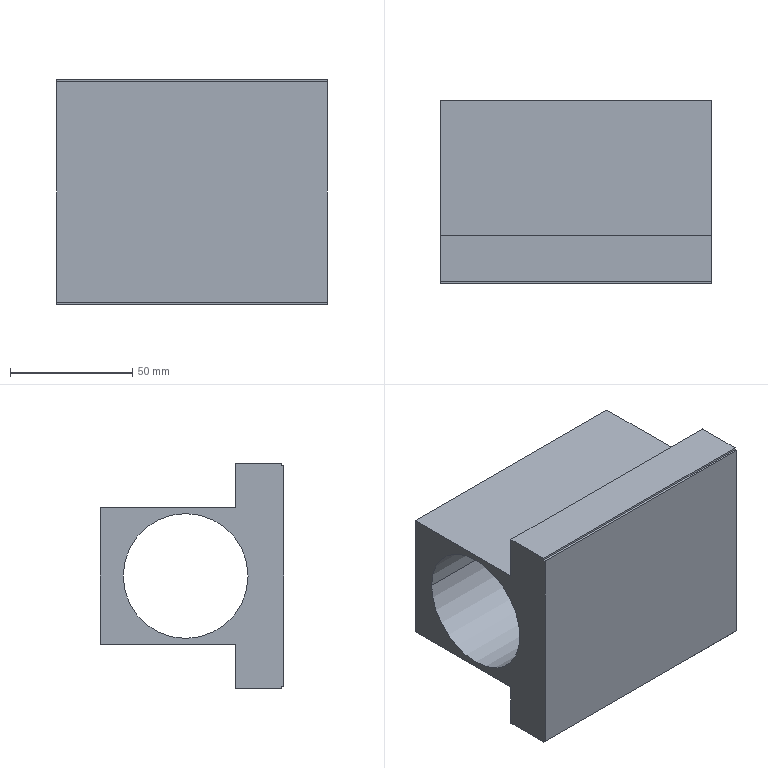Component | SolidWorks | ConnectingSeat-1 | 1 solid | 34 faces | box 111 x 75.24 x 92.14 mm | volume 314296 mm3 | plane 20 | cylinder 14 | commonest cylinder face diameters 8 x8 5.551 x4 51.14 x2
build123d program:
from build123d import *

# Parameters (mm, degrees)
BOSS_EXTRUDE1_DEPTH  = 111
SKETCH4_R            = 18.564
CUT_EXTRUDE1_2_DEPTH = 111
SKETCH5_W            = 55.24
SKETCH5_H            = 35.775
CUT_EXTRUDE2_DEPTH   = 171
SKETCH6_R            = 25.57
CUT_EXTRUDE3_DEPTH   = 115
SKETCH7_R            = 25.57
BOSS_EXTRUDE2_DEPTH  = 111
SKETCH9_R            = 4
CUT_EXTRUDE4_DEPTH   = 13.5
SKETCH10_R           = 2.776
CUT_EXTRUDE5_DEPTH   = 13.5
SKETCH1_W            = 1
SKETCH1_H            = 1.15
CUT_EXTRUDE1_DEPTH   = 133.269


with BuildPart() as part:
    # Sketch3 → Boss-Extrude1 (new body)
    with BuildSketch(Plane.ZY.offset(277)):
        Polygon((-20, -46.072), (-20, 46.072), (-0.1784, 46.072), (-0.1784, 27.887), (55.24, 27.887), (55.24, -27.887), (-0.1784, -27.887), (-0.1784, -46.072), align=None)
    extrude(amount=-BOSS_EXTRUDE1_DEPTH)

    # Sketch4 → Cut-Extrude1_2 (cut)
    with BuildSketch(Plane.ZY.offset(277)):
        with Locations((20.219, 0)):
            Circle(SKETCH4_R)
    extrude(amount=-CUT_EXTRUDE1_2_DEPTH, mode=Mode.SUBTRACT)

    # Sketch5 → Cut-Extrude2 (cut)
    with BuildSketch(Plane(origin=(-166, 0, 0), x_dir=(0, 0, -1), z_dir=(1, 0, 0))):
        with Locations((-17.62, 0)):
            Rectangle(SKETCH5_W, SKETCH5_H)
    extrude(amount=-CUT_EXTRUDE2_DEPTH, mode=Mode.SUBTRACT)

    # Sketch6 → Cut-Extrude3 (cut)
    with BuildSketch(Plane(origin=(-166, 0, 0), x_dir=(0, 0, -1), z_dir=(1, 0, 0))):
        with Locations((-20.219, 0)):
            Circle(SKETCH6_R)
    extrude(amount=-CUT_EXTRUDE3_DEPTH, mode=Mode.SUBTRACT)

    # Sketch7 → Boss-Extrude2 (add)
    with BuildSketch(Plane(origin=(-166, 0, 0), x_dir=(0, 0, -1), z_dir=(1, 0, 0))):
        Polygon((-55.24, 27.887), (-55.24, -27.887), (0.1784, -27.887), (0.1784, -46.072), (20, -46.072), (20, 46.072), (0.1784, 46.072), (0.1784, 27.887), align=None)
        with Locations((-20.219, 0)):
            Circle(SKETCH7_R, mode=Mode.SUBTRACT)
    extrude(amount=-BOSS_EXTRUDE2_DEPTH)

    # Sketch9 → Cut-Extrude4 (cut)
    with BuildSketch(Plane.XY.offset(-0.1784)):
        with Locations((-256.037, 36.566)):
            Circle(SKETCH9_R)
        with Locations((-186.382, 36.566)):
            Circle(SKETCH9_R)
        with Locations(Location((-186.382, -36.566, 0), (0, 0, 180))):
            Circle(SKETCH9_R)
        with Locations(Location((-256.037, -36.566, 0), (0, 0, 180))):
            Circle(SKETCH9_R)
    extrude(amount=-CUT_EXTRUDE4_DEPTH, mode=Mode.SUBTRACT)

    # Sketch10 → Cut-Extrude5 (cut)
    with BuildSketch(Plane.XY.offset(-0.1784)):
        with Locations((-221.326, 36.732)):
            Circle(SKETCH10_R)
        with Locations(Location((-221.326, -36.732, 0), (0, 0, 180))):
            Circle(SKETCH10_R)
    extrude(amount=-CUT_EXTRUDE5_DEPTH, mode=Mode.SUBTRACT)

    # Sketch1 → Cut-Extrude1 (cut, through all)
    with BuildSketch(Plane(origin=(-166, 0, 0), x_dir=(0, 0, -1), z_dir=(1, 0, 0))):
        with Locations((19.6, -45.825)):
            Rectangle(SKETCH1_W, SKETCH1_H)
        with Locations((19.6, 45.825)):
            Rectangle(SKETCH1_W, SKETCH1_H)
    extrude(amount=-CUT_EXTRUDE1_DEPTH, mode=Mode.SUBTRACT)


solid = part.part

# Placed as in the assembly
solid = solid.moved(Location((0, 40, 0), (-90, 0, 0)))
STEP:
#1=CARTESIAN_POINT('',(-8.823,1.036,1.446));
#2=VERTEX_POINT('',#1);
#3=CARTESIAN_POINT('',(-8.604,1.036,1.446));
#4=VERTEX_POINT('',#3);
#5=CARTESIAN_POINT('',(-8.714,1.036,1.446));
#6=DIRECTION('',(0.,1.,0.));
#7=DIRECTION('',(-1.,0.,0.));
#8=AXIS2_PLACEMENT_3D('',#5,#6,#7);
#9=CIRCLE('',#8,0.1093);
#10=EDGE_CURVE('',#2,#4,#9,.T.);
#11=ORIENTED_EDGE('',*,*,#10,.F.);
#12=CARTESIAN_POINT('',(-8.823,1.568,1.446));
#13=VERTEX_POINT('',#12);
#14=CARTESIAN_POINT('',(-8.823,1.036,1.446));
#15=DIRECTION('',(0.,1.,0.));
#16=VECTOR('',#15,39.37);
#17=LINE('',#14,#16);
#18=EDGE_CURVE('',#2,#13,#17,.T.);
#19=ORIENTED_EDGE('',*,*,#18,.T.);
#20=CARTESIAN_POINT('',(-8.604,1.568,1.446));
#21=VERTEX_POINT('',#20);
#22=CARTESIAN_POINT('',(-8.714,1.568,1.446));
#23=DIRECTION('',(0.,1.,0.));
#24=DIRECTION('',(-1.,0.,0.));
#25=AXIS2_PLACEMENT_3D('',#22,#23,#24);
#26=CIRCLE('',#25,0.1093);
#27=EDGE_CURVE('',#13,#21,#26,.T.);
#28=ORIENTED_EDGE('',*,*,#27,.T.);
#29=CARTESIAN_POINT('',(-8.604,1.036,1.446));
#30=DIRECTION('',(0.,1.,0.));
#31=VECTOR('',#30,39.37);
#32=LINE('',#29,#31);
#33=EDGE_CURVE('',#4,#21,#32,.T.);
#34=ORIENTED_EDGE('',*,*,#33,.F.);
#35=EDGE_LOOP('',(#11,#19,#28,#34));
#36=FACE_OUTER_BOUND('',#35,.T.);
#37=CARTESIAN_POINT('',(-8.714,1.036,1.446));
#38=DIRECTION('',(0.,1.,0.));
#39=DIRECTION('',(1.,0.,0.));
#40=AXIS2_PLACEMENT_3D('',#37,#38,#39);
#41=CYLINDRICAL_SURFACE('',#40,0.1093);
#42=ADVANCED_FACE('',(#36),#41,.F.);
#43=CARTESIAN_POINT('',(-8.823,1.036,-1.446));
#44=VERTEX_POINT('',#43);
#45=CARTESIAN_POINT('',(-8.604,1.036,-1.446));
#46=VERTEX_POINT('',#45);
#47=CARTESIAN_POINT('',(-8.714,1.036,-1.446));
#48=DIRECTION('',(0.,1.,0.));
#49=DIRECTION('',(1.,0.,0.));
#50=AXIS2_PLACEMENT_3D('',#47,#48,#49);
#51=CIRCLE('',#50,0.1093);
#52=EDGE_CURVE('',#44,#46,#51,.T.);
#53=ORIENTED_EDGE('',*,*,#52,.F.);
#54=CARTESIAN_POINT('',(-8.823,1.568,-1.446));
#55=VERTEX_POINT('',#54);
#56=CARTESIAN_POINT('',(-8.823,1.036,-1.446));
#57=DIRECTION('',(0.,1.,0.));
#58=VECTOR('',#57,39.37);
#59=LINE('',#56,#58);
#60=EDGE_CURVE('',#44,#55,#59,.T.);
#61=ORIENTED_EDGE('',*,*,#60,.T.);
#62=CARTESIAN_POINT('',(-8.604,1.568,-1.446));
#63=VERTEX_POINT('',#62);
#64=CARTESIAN_POINT('',(-8.714,1.568,-1.446));
#65=DIRECTION('',(0.,1.,0.));
#66=DIRECTION('',(1.,0.,0.));
#67=AXIS2_PLACEMENT_3D('',#64,#65,#66);
#68=CIRCLE('',#67,0.1093);
#69=EDGE_CURVE('',#55,#63,#68,.T.);
#70=ORIENTED_EDGE('',*,*,#69,.T.);
#71=CARTESIAN_POINT('',(-8.604,1.036,-1.446));
#72=DIRECTION('',(0.,1.,0.));
#73=VECTOR('',#72,39.37);
#74=LINE('',#71,#73);
#75=EDGE_CURVE('',#46,#63,#74,.T.);
#76=ORIENTED_EDGE('',*,*,#75,.F.);
#77=EDGE_LOOP('',(#53,#61,#70,#76));
#78=FACE_OUTER_BOUND('',#77,.T.);
#79=CARTESIAN_POINT('',(-8.714,1.036,-1.446));
#80=DIRECTION('',(0.,1.,0.));
#81=DIRECTION('',(1.,0.,0.));
#82=AXIS2_PLACEMENT_3D('',#79,#80,#81);
#83=CYLINDRICAL_SURFACE('',#82,0.1093);
#84=ADVANCED_FACE('',(#78),#83,.F.);
#85=CARTESIAN_POINT('',(-10.238,1.036,1.44));
#86=VERTEX_POINT('',#85);
#87=CARTESIAN_POINT('',(-9.923,1.036,1.44));
#88=VERTEX_POINT('',#87);
#89=CARTESIAN_POINT('',(-10.08,1.036,1.44));
#90=DIRECTION('',(0.,1.,0.));
#91=DIRECTION('',(-1.,0.,0.));
#92=AXIS2_PLACEMENT_3D('',#89,#90,#91);
#93=CIRCLE('',#92,0.1575);
#94=EDGE_CURVE('',#86,#88,#93,.T.);
#95=ORIENTED_EDGE('',*,*,#94,.F.);
#96=CARTESIAN_POINT('',(-10.238,1.568,1.44));
#97=VERTEX_POINT('',#96);
#98=CARTESIAN_POINT('',(-10.238,1.036,1.44));
#99=DIRECTION('',(0.,1.,0.));
#100=VECTOR('',#99,39.37);
#101=LINE('',#98,#100);
#102=EDGE_CURVE('',#86,#97,#101,.T.);
#103=ORIENTED_EDGE('',*,*,#102,.T.);
#104=CARTESIAN_POINT('',(-9.923,1.568,1.44));
#105=VERTEX_POINT('',#104);
#106=CARTESIAN_POINT('',(-10.08,1.568,1.44));
#107=DIRECTION('',(0.,1.,0.));
#108=DIRECTION('',(-1.,0.,0.));
#109=AXIS2_PLACEMENT_3D('',#106,#107,#108);
#110=CIRCLE('',#109,0.1575);
#111=EDGE_CURVE('',#97,#105,#110,.T.);
#112=ORIENTED_EDGE('',*,*,#111,.T.);
#113=CARTESIAN_POINT('',(-9.923,1.036,1.44));
#114=DIRECTION('',(0.,1.,0.));
#115=VECTOR('',#114,39.37);
#116=LINE('',#113,#115);
#117=EDGE_CURVE('',#88,#105,#116,.T.);
#118=ORIENTED_EDGE('',*,*,#117,.F.);
#119=EDGE_LOOP('',(#95,#103,#112,#118));
#120=FACE_OUTER_BOUND('',#119,.T.);
#121=CARTESIAN_POINT('',(-10.08,1.036,1.44));
#122=DIRECTION('',(0.,1.,0.));
#123=DIRECTION('',(1.,0.,0.));
#124=AXIS2_PLACEMENT_3D('',#121,#122,#123);
#125=CYLINDRICAL_SURFACE('',#124,0.1575);
#126=ADVANCED_FACE('',(#120),#125,.F.);
#127=CARTESIAN_POINT('',(-7.495,1.036,1.44));
#128=VERTEX_POINT('',#127);
#129=CARTESIAN_POINT('',(-7.18,1.036,1.44));
#130=VERTEX_POINT('',#129);
#131=CARTESIAN_POINT('',(-7.338,1.036,1.44));
#132=DIRECTION('',(0.,1.,0.));
#133=DIRECTION('',(-1.,0.,0.));
#134=AXIS2_PLACEMENT_3D('',#131,#132,#133);
#135=CIRCLE('',#134,0.1575);
#136=EDGE_CURVE('',#128,#130,#135,.T.);
#137=ORIENTED_EDGE('',*,*,#136,.F.);
#138=CARTESIAN_POINT('',(-7.495,1.568,1.44));
#139=VERTEX_POINT('',#138);
#140=CARTESIAN_POINT('',(-7.495,1.036,1.44));
#141=DIRECTION('',(0.,1.,0.));
#142=VECTOR('',#141,39.37);
#143=LINE('',#140,#142);
#144=EDGE_CURVE('',#128,#139,#143,.T.);
#145=ORIENTED_EDGE('',*,*,#144,.T.);
#146=CARTESIAN_POINT('',(-7.18,1.568,1.44));
#147=VERTEX_POINT('',#146);
#148=CARTESIAN_POINT('',(-7.338,1.568,1.44));
#149=DIRECTION('',(0.,1.,0.));
#150=DIRECTION('',(-1.,0.,0.));
#151=AXIS2_PLACEMENT_3D('',#148,#149,#150);
#152=CIRCLE('',#151,0.1575);
#153=EDGE_CURVE('',#139,#147,#152,.T.);
#154=ORIENTED_EDGE('',*,*,#153,.T.);
#155=CARTESIAN_POINT('',(-7.18,1.036,1.44));
#156=DIRECTION('',(0.,1.,0.));
#157=VECTOR('',#156,39.37);
#158=LINE('',#155,#157);
#159=EDGE_CURVE('',#130,#147,#158,.T.);
#160=ORIENTED_EDGE('',*,*,#159,.F.);
#161=EDGE_LOOP('',(#137,#145,#154,#160));
#162=FACE_OUTER_BOUND('',#161,.T.);
#163=CARTESIAN_POINT('',(-7.338,1.036,1.44));
#164=DIRECTION('',(0.,1.,0.));
#165=DIRECTION('',(1.,0.,0.));
#166=AXIS2_PLACEMENT_3D('',#163,#164,#165);
#167=CYLINDRICAL_SURFACE('',#166,0.1575);
#168=ADVANCED_FACE('',(#162),#167,.F.);
#169=CARTESIAN_POINT('',(-7.495,1.036,-1.44));
#170=VERTEX_POINT('',#169);
#171=CARTESIAN_POINT('',(-7.18,1.036,-1.44));
#172=VERTEX_POINT('',#171);
#173=CARTESIAN_POINT('',(-7.338,1.036,-1.44));
#174=DIRECTION('',(0.,1.,0.));
#175=DIRECTION('',(1.,0.,0.));
#176=AXIS2_PLACEMENT_3D('',#173,#174,#175);
#177=CIRCLE('',#176,0.1575);
#178=EDGE_CURVE('',#170,#172,#177,.T.);
#179=ORIENTED_EDGE('',*,*,#178,.F.);
#180=CARTESIAN_POINT('',(-7.495,1.568,-1.44));
#181=VERTEX_POINT('',#180);
#182=CARTESIAN_POINT('',(-7.495,1.036,-1.44));
#183=DIRECTION('',(0.,1.,0.));
#184=VECTOR('',#183,39.37);
#185=LINE('',#182,#184);
#186=EDGE_CURVE('',#170,#181,#185,.T.);
#187=ORIENTED_EDGE('',*,*,#186,.T.);
#188=CARTESIAN_POINT('',(-7.18,1.568,-1.44));
#189=VERTEX_POINT('',#188);
#190=CARTESIAN_POINT('',(-7.338,1.568,-1.44));
#191=DIRECTION('',(0.,1.,0.));
#192=DIRECTION('',(1.,0.,0.));
#193=AXIS2_PLACEMENT_3D('',#190,#191,#192);
#194=CIRCLE('',#193,0.1575);
#195=EDGE_CURVE('',#181,#189,#194,.T.);
#196=ORIENTED_EDGE('',*,*,#195,.T.);
#197=CARTESIAN_POINT('',(-7.18,1.036,-1.44));
#198=DIRECTION('',(0.,1.,0.));
#199=VECTOR('',#198,39.37);
#200=LINE('',#197,#199);
#201=EDGE_CURVE('',#172,#189,#200,.T.);
#202=ORIENTED_EDGE('',*,*,#201,.F.);
#203=EDGE_LOOP('',(#179,#187,#196,#202));
#204=FACE_OUTER_BOUND('',#203,.T.);
#205=CARTESIAN_POINT('',(-7.338,1.036,-1.44));
#206=DIRECTION('',(0.,1.,0.));
#207=DIRECTION('',(1.,0.,0.));
#208=AXIS2_PLACEMENT_3D('',#205,#206,#207);
#209=CYLINDRICAL_SURFACE('',#208,0.1575);
#210=ADVANCED_FACE('',(#204),#209,.F.);
#211=CARTESIAN_POINT('',(-10.238,1.036,-1.44));
#212=VERTEX_POINT('',#211);
#213=CARTESIAN_POINT('',(-9.923,1.036,-1.44));
#214=VERTEX_POINT('',#213);
#215=CARTESIAN_POINT('',(-10.08,1.036,-1.44));
#216=DIRECTION('',(0.,1.,0.));
#217=DIRECTION('',(1.,0.,0.));
#218=AXIS2_PLACEMENT_3D('',#215,#216,#217);
#219=CIRCLE('',#218,0.1575);
#220=EDGE_CURVE('',#212,#214,#219,.T.);
#221=ORIENTED_EDGE('',*,*,#220,.F.);
#222=CARTESIAN_POINT('',(-10.238,1.568,-1.44));
#223=VERTEX_POINT('',#222);
#224=CARTESIAN_POINT('',(-10.238,1.036,-1.44));
#225=DIRECTION('',(0.,1.,0.));
#226=VECTOR('',#225,39.37);
#227=LINE('',#224,#226);
#228=EDGE_CURVE('',#212,#223,#227,.T.);
#229=ORIENTED_EDGE('',*,*,#228,.T.);
#230=CARTESIAN_POINT('',(-9.923,1.568,-1.44));
#231=VERTEX_POINT('',#230);
#232=CARTESIAN_POINT('',(-10.08,1.568,-1.44));
#233=DIRECTION('',(0.,1.,0.));
#234=DIRECTION('',(1.,0.,0.));
#235=AXIS2_PLACEMENT_3D('',#232,#233,#234);
#236=CIRCLE('',#235,0.1575);
#237=EDGE_CURVE('',#223,#231,#236,.T.);
#238=ORIENTED_EDGE('',*,*,#237,.T.);
#239=CARTESIAN_POINT('',(-9.923,1.036,-1.44));
#240=DIRECTION('',(0.,1.,0.));
#241=VECTOR('',#240,39.37);
#242=LINE('',#239,#241);
#243=EDGE_CURVE('',#214,#231,#242,.T.);
#244=ORIENTED_EDGE('',*,*,#243,.F.);
#245=EDGE_LOOP('',(#221,#229,#238,#244));
#246=FACE_OUTER_BOUND('',#245,.T.);
#247=CARTESIAN_POINT('',(-10.08,1.036,-1.44));
#248=DIRECTION('',(0.,1.,0.));
#249=DIRECTION('',(1.,0.,0.));
#250=AXIS2_PLACEMENT_3D('',#247,#248,#249);
#251=CYLINDRICAL_SURFACE('',#250,0.1575);
#252=ADVANCED_FACE('',(#246),#251,.F.);
#253=CARTESIAN_POINT('',(-10.906,1.364,0.));
#254=VERTEX_POINT('',#253);
#255=CARTESIAN_POINT('',(-10.906,3.378,0.));
#256=VERTEX_POINT('',#255);
#257=CARTESIAN_POINT('',(-10.906,2.371,0.));
#258=DIRECTION('',(-1.,0.,0.));
#259=DIRECTION('',(0.,1.,0.));
#260=AXIS2_PLACEMENT_3D('',#257,#258,#259);
#261=CIRCLE('',#260,1.007);
#262=EDGE_CURVE('',#254,#256,#261,.T.);
#263=ORIENTED_EDGE('',*,*,#262,.T.);
#264=CARTESIAN_POINT('',(-6.535,3.378,0.));
#265=VERTEX_POINT('',#264);
#266=CARTESIAN_POINT('',(-11.063,3.378,0.));
#267=DIRECTION('',(1.,0.,0.));
#268=VECTOR('',#267,39.37);
#269=LINE('',#266,#268);
#270=EDGE_CURVE('',#256,#265,#269,.T.);
#271=ORIENTED_EDGE('',*,*,#270,.T.);
#272=CARTESIAN_POINT('',(-6.535,1.364,0.));
#273=VERTEX_POINT('',#272);
#274=CARTESIAN_POINT('',(-6.535,2.371,0.));
#275=DIRECTION('',(1.,0.,0.));
#276=DIRECTION('',(0.,-1.,0.));
#277=AXIS2_PLACEMENT_3D('',#274,#275,#276);
#278=CIRCLE('',#277,1.007);
#279=EDGE_CURVE('',#265,#273,#278,.T.);
#280=ORIENTED_EDGE('',*,*,#279,.T.);
#281=CARTESIAN_POINT('',(-11.063,1.364,0.));
#282=DIRECTION('',(1.,0.,0.));
#283=VECTOR('',#282,39.37);
#284=LINE('',#281,#283);
#285=EDGE_CURVE('',#254,#273,#284,.T.);
#286=ORIENTED_EDGE('',*,*,#285,.F.);
#287=EDGE_LOOP('',(#263,#271,#280,#286));
#288=FACE_OUTER_BOUND('',#287,.T.);
#289=CARTESIAN_POINT('',(-11.063,2.371,0.));
#290=DIRECTION('',(1.,0.,0.));
#291=DIRECTION('',(0.,-1.,0.));
#292=AXIS2_PLACEMENT_3D('',#289,#290,#291);
#293=CYLINDRICAL_SURFACE('',#292,1.007);
#294=ADVANCED_FACE('',(#288),#293,.F.);
#295=CARTESIAN_POINT('',(-6.535,2.371,0.));
#296=DIRECTION('',(1.,0.,0.));
#297=DIRECTION('',(0.,-1.,0.));
#298=AXIS2_PLACEMENT_3D('',#295,#296,#297);
#299=CIRCLE('',#298,1.007);
#300=EDGE_CURVE('',#273,#265,#299,.T.);
#301=ORIENTED_EDGE('',*,*,#300,.F.);
#302=ORIENTED_EDGE('',*,*,#279,.F.);
#303=EDGE_LOOP('',(#301,#302));
#304=FACE_BOUND('',#303,.T.);
#305=CARTESIAN_POINT('',(-6.535,0.7874,1.781));
#306=VERTEX_POINT('',#305);
#307=CARTESIAN_POINT('',(-6.535,0.8228,1.781));
#308=VERTEX_POINT('',#307);
#309=CARTESIAN_POINT('',(-6.535,0.7835,1.781));
#310=DIRECTION('',(0.,1.,0.));
#311=VECTOR('',#310,39.37);
#312=LINE('',#309,#311);
#313=EDGE_CURVE('',#306,#308,#312,.T.);
#314=ORIENTED_EDGE('',*,*,#313,.F.);
#315=CARTESIAN_POINT('',(-6.535,0.7874,-1.781));
#316=VERTEX_POINT('',#315);
#317=CARTESIAN_POINT('',(-6.535,0.7874,1.814));
#318=DIRECTION('',(0.,-0.,1.));
#319=VECTOR('',#318,39.37);
#320=LINE('',#317,#319);
#321=EDGE_CURVE('',#316,#306,#320,.T.);
#322=ORIENTED_EDGE('',*,*,#321,.F.);
#323=CARTESIAN_POINT('',(-6.535,0.8228,-1.781));
#324=VERTEX_POINT('',#323);
#325=CARTESIAN_POINT('',(-6.535,0.7835,-1.781));
#326=DIRECTION('',(0.,-1.,0.));
#327=VECTOR('',#326,39.37);
#328=LINE('',#325,#327);
#329=EDGE_CURVE('',#324,#316,#328,.T.);
#330=ORIENTED_EDGE('',*,*,#329,.F.);
#331=CARTESIAN_POINT('',(-6.535,0.8228,-1.814));
#332=VERTEX_POINT('',#331);
#333=CARTESIAN_POINT('',(-6.535,0.8228,-1.827));
#334=DIRECTION('',(0.,0.,1.));
#335=VECTOR('',#334,39.37);
#336=LINE('',#333,#335);
#337=EDGE_CURVE('',#332,#324,#336,.T.);
#338=ORIENTED_EDGE('',*,*,#337,.F.);
#339=CARTESIAN_POINT('',(-6.535,1.568,-1.814));
#340=VERTEX_POINT('',#339);
#341=CARTESIAN_POINT('',(-6.535,0.7874,-1.814));
#342=DIRECTION('',(0.,-1.,0.));
#343=VECTOR('',#342,39.37);
#344=LINE('',#341,#343);
#345=EDGE_CURVE('',#340,#332,#344,.T.);
#346=ORIENTED_EDGE('',*,*,#345,.F.);
#347=CARTESIAN_POINT('',(-6.535,1.568,-1.098));
#348=VERTEX_POINT('',#347);
#349=CARTESIAN_POINT('',(-6.535,1.568,-1.814));
#350=DIRECTION('',(0.,0.,-1.));
#351=VECTOR('',#350,39.37);
#352=LINE('',#349,#351);
#353=EDGE_CURVE('',#348,#340,#352,.T.);
#354=ORIENTED_EDGE('',*,*,#353,.F.);
#355=CARTESIAN_POINT('',(-6.535,3.75,-1.098));
#356=VERTEX_POINT('',#355);
#357=CARTESIAN_POINT('',(-6.535,1.568,-1.098));
#358=DIRECTION('',(0.,-1.,0.));
#359=VECTOR('',#358,39.37);
#360=LINE('',#357,#359);
#361=EDGE_CURVE('',#356,#348,#360,.T.);
#362=ORIENTED_EDGE('',*,*,#361,.F.);
#363=CARTESIAN_POINT('',(-6.535,3.75,1.098));
#364=VERTEX_POINT('',#363);
#365=CARTESIAN_POINT('',(-6.535,3.75,-1.098));
#366=DIRECTION('',(0.,0.,-1.));
#367=VECTOR('',#366,39.37);
#368=LINE('',#365,#367);
#369=EDGE_CURVE('',#364,#356,#368,.T.);
#370=ORIENTED_EDGE('',*,*,#369,.F.);
#371=CARTESIAN_POINT('',(-6.535,1.568,1.098));
#372=VERTEX_POINT('',#371);
#373=CARTESIAN_POINT('',(-6.535,1.568,1.098));
#374=DIRECTION('',(0.,1.,0.));
#375=VECTOR('',#374,39.37);
#376=LINE('',#373,#375);
#377=EDGE_CURVE('',#372,#364,#376,.T.);
#378=ORIENTED_EDGE('',*,*,#377,.F.);
#379=CARTESIAN_POINT('',(-6.535,1.568,1.814));
#380=VERTEX_POINT('',#379);
#381=CARTESIAN_POINT('',(-6.535,1.568,1.814));
#382=DIRECTION('',(0.,0.,-1.));
#383=VECTOR('',#382,39.37);
#384=LINE('',#381,#383);
#385=EDGE_CURVE('',#380,#372,#384,.T.);
#386=ORIENTED_EDGE('',*,*,#385,.F.);
#387=CARTESIAN_POINT('',(-6.535,0.8228,1.814));
#388=VERTEX_POINT('',#387);
#389=CARTESIAN_POINT('',(-6.535,0.7874,1.814));
#390=DIRECTION('',(0.,1.,0.));
#391=VECTOR('',#390,39.37);
#392=LINE('',#389,#391);
#393=EDGE_CURVE('',#388,#380,#392,.T.);
#394=ORIENTED_EDGE('',*,*,#393,.F.);
#395=CARTESIAN_POINT('',(-6.535,0.8228,1.781));
#396=DIRECTION('',(0.,0.,1.));
#397=VECTOR('',#396,39.37);
#398=LINE('',#395,#397);
#399=EDGE_CURVE('',#308,#388,#398,.T.);
#400=ORIENTED_EDGE('',*,*,#399,.F.);
#401=EDGE_LOOP('',(#314,#322,#330,#338,#346,#354,#362,#370,#378,#386,#394,#400));
#402=FACE_OUTER_BOUND('',#401,.T.);
#403=CARTESIAN_POINT('',(-6.535,1.575,0.));
#404=DIRECTION('',(-1.,0.,0.));
#405=DIRECTION('',(0.,1.,0.));
#406=AXIS2_PLACEMENT_3D('',#403,#404,#405);
#407=PLANE('',#406);
#408=ADVANCED_FACE('',(#304,#402),#407,.F.);
#409=ORIENTED_EDGE('',*,*,#262,.F.);
#410=CARTESIAN_POINT('',(-10.906,2.371,0.));
#411=DIRECTION('',(-1.,0.,0.));
#412=DIRECTION('',(0.,1.,0.));
#413=AXIS2_PLACEMENT_3D('',#410,#411,#412);
#414=CIRCLE('',#413,1.007);
#415=EDGE_CURVE('',#256,#254,#414,.T.);
#416=ORIENTED_EDGE('',*,*,#415,.F.);
#417=EDGE_LOOP('',(#409,#416));
#418=FACE_BOUND('',#417,.T.);
#419=CARTESIAN_POINT('',(-10.906,0.7874,1.781));
#420=VERTEX_POINT('',#419);
#421=CARTESIAN_POINT('',(-10.906,0.8228,1.781));
#422=VERTEX_POINT('',#421);
#423=CARTESIAN_POINT('',(-10.906,0.7835,1.781));
#424=DIRECTION('',(0.,1.,0.));
#425=VECTOR('',#424,39.37);
#426=LINE('',#423,#425);
#427=EDGE_CURVE('',#420,#422,#426,.T.);
#428=ORIENTED_EDGE('',*,*,#427,.T.);
#429=CARTESIAN_POINT('',(-10.906,0.8228,1.814));
#430=VERTEX_POINT('',#429);
#431=CARTESIAN_POINT('',(-10.906,0.8228,1.781));
#432=DIRECTION('',(0.,0.,1.));
#433=VECTOR('',#432,39.37);
#434=LINE('',#431,#433);
#435=EDGE_CURVE('',#422,#430,#434,.T.);
#436=ORIENTED_EDGE('',*,*,#435,.T.);
#437=CARTESIAN_POINT('',(-10.906,1.568,1.814));
#438=VERTEX_POINT('',#437);
#439=CARTESIAN_POINT('',(-10.906,0.7874,1.814));
#440=DIRECTION('',(0.,1.,0.));
#441=VECTOR('',#440,39.37);
#442=LINE('',#439,#441);
#443=EDGE_CURVE('',#430,#438,#442,.T.);
#444=ORIENTED_EDGE('',*,*,#443,.T.);
#445=CARTESIAN_POINT('',(-10.906,1.568,1.098));
#446=VERTEX_POINT('',#445);
#447=CARTESIAN_POINT('',(-10.906,1.568,1.814));
#448=DIRECTION('',(0.,0.,-1.));
#449=VECTOR('',#448,39.37);
#450=LINE('',#447,#449);
#451=EDGE_CURVE('',#438,#446,#450,.T.);
#452=ORIENTED_EDGE('',*,*,#451,.T.);
#453=CARTESIAN_POINT('',(-10.906,3.75,1.098));
#454=VERTEX_POINT('',#453);
#455=CARTESIAN_POINT('',(-10.906,1.568,1.098));
#456=DIRECTION('',(0.,1.,0.));
#457=VECTOR('',#456,39.37);
#458=LINE('',#455,#457);
#459=EDGE_CURVE('',#446,#454,#458,.T.);
#460=ORIENTED_EDGE('',*,*,#459,.T.);
#461=CARTESIAN_POINT('',(-10.906,3.75,-1.098));
#462=VERTEX_POINT('',#461);
#463=CARTESIAN_POINT('',(-10.906,3.75,-1.098));
#464=DIRECTION('',(0.,0.,-1.));
#465=VECTOR('',#464,39.37);
#466=LINE('',#463,#465);
#467=EDGE_CURVE('',#454,#462,#466,.T.);
#468=ORIENTED_EDGE('',*,*,#467,.T.);
#469=CARTESIAN_POINT('',(-10.906,1.568,-1.098));
#470=VERTEX_POINT('',#469);
#471=CARTESIAN_POINT('',(-10.906,1.568,-1.098));
#472=DIRECTION('',(0.,-1.,0.));
#473=VECTOR('',#472,39.37);
#474=LINE('',#471,#473);
#475=EDGE_CURVE('',#462,#470,#474,.T.);
#476=ORIENTED_EDGE('',*,*,#475,.T.);
#477=CARTESIAN_POINT('',(-10.906,1.568,-1.814));
#478=VERTEX_POINT('',#477);
#479=CARTESIAN_POINT('',(-10.906,1.568,-1.814));
#480=DIRECTION('',(0.,0.,-1.));
#481=VECTOR('',#480,39.37);
#482=LINE('',#479,#481);
#483=EDGE_CURVE('',#470,#478,#482,.T.);
#484=ORIENTED_EDGE('',*,*,#483,.T.);
#485=CARTESIAN_POINT('',(-10.906,0.8228,-1.814));
#486=VERTEX_POINT('',#485);
#487=CARTESIAN_POINT('',(-10.906,0.7874,-1.814));
#488=DIRECTION('',(0.,-1.,0.));
#489=VECTOR('',#488,39.37);
#490=LINE('',#487,#489);
#491=EDGE_CURVE('',#478,#486,#490,.T.);
#492=ORIENTED_EDGE('',*,*,#491,.T.);
#493=CARTESIAN_POINT('',(-10.906,0.8228,-1.781));
#494=VERTEX_POINT('',#493);
#495=CARTESIAN_POINT('',(-10.906,0.8228,-1.827));
#496=DIRECTION('',(0.,0.,1.));
#497=VECTOR('',#496,39.37);
#498=LINE('',#495,#497);
#499=EDGE_CURVE('',#486,#494,#498,.T.);
#500=ORIENTED_EDGE('',*,*,#499,.T.);
#501=CARTESIAN_POINT('',(-10.906,0.7874,-1.781));
#502=VERTEX_POINT('',#501);
#503=CARTESIAN_POINT('',(-10.906,0.7835,-1.781));
#504=DIRECTION('',(0.,-1.,0.));
#505=VECTOR('',#504,39.37);
#506=LINE('',#503,#505);
#507=EDGE_CURVE('',#494,#502,#506,.T.);
#508=ORIENTED_EDGE('',*,*,#507,.T.);
#509=CARTESIAN_POINT('',(-10.906,0.7874,1.814));
#510=DIRECTION('',(0.,-0.,1.));
#511=VECTOR('',#510,39.37);
#512=LINE('',#509,#511);
#513=EDGE_CURVE('',#502,#420,#512,.T.);
#514=ORIENTED_EDGE('',*,*,#513,.T.);
#515=EDGE_LOOP('',(#428,#436,#444,#452,#460,#468,#476,#484,#492,#500,#508,#514));
#516=FACE_OUTER_BOUND('',#515,.T.);
#517=CARTESIAN_POINT('',(-10.906,1.575,0.));
#518=DIRECTION('',(-1.,0.,0.));
#519=DIRECTION('',(0.,1.,0.));
#520=AXIS2_PLACEMENT_3D('',#517,#518,#519);
#521=PLANE('',#520);
#522=ADVANCED_FACE('',(#418,#516),#521,.T.);
#523=ORIENTED_EDGE('',*,*,#467,.F.);
#524=CARTESIAN_POINT('',(-6.535,3.75,1.098));
#525=DIRECTION('',(-1.,0.,0.));
#526=VECTOR('',#525,39.37);
#527=LINE('',#524,#526);
#528=EDGE_CURVE('',#364,#454,#527,.T.);
#529=ORIENTED_EDGE('',*,*,#528,.F.);
#530=ORIENTED_EDGE('',*,*,#369,.T.);
#531=CARTESIAN_POINT('',(-6.535,3.75,-1.098));
#532=DIRECTION('',(-1.,0.,0.));
#533=VECTOR('',#532,39.37);
#534=LINE('',#531,#533);
#535=EDGE_CURVE('',#356,#462,#534,.T.);
#536=ORIENTED_EDGE('',*,*,#535,.T.);
#537=EDGE_LOOP('',(#523,#529,#530,#536));
#538=FACE_OUTER_BOUND('',#537,.T.);
#539=CARTESIAN_POINT('',(-6.535,3.75,-1.098));
#540=DIRECTION('',(0.,1.,0.));
#541=DIRECTION('',(1.,0.,0.));
#542=AXIS2_PLACEMENT_3D('',#539,#540,#541);
#543=PLANE('',#542);
#544=ADVANCED_FACE('',(#538),#543,.T.);
#545=ORIENTED_EDGE('',*,*,#459,.F.);
#546=CARTESIAN_POINT('',(-6.535,1.568,1.098));
#547=DIRECTION('',(-1.,0.,0.));
#548=VECTOR('',#547,39.37);
#549=LINE('',#546,#548);
#550=EDGE_CURVE('',#372,#446,#549,.T.);
#551=ORIENTED_EDGE('',*,*,#550,.F.);
#552=ORIENTED_EDGE('',*,*,#377,.T.);
#553=ORIENTED_EDGE('',*,*,#528,.T.);
#554=EDGE_LOOP('',(#545,#551,#552,#553));
#555=FACE_OUTER_BOUND('',#554,.T.);
#556=CARTESIAN_POINT('',(-6.535,1.568,1.098));
#557=DIRECTION('',(0.,0.,1.));
#558=DIRECTION('',(0.,-1.,0.));
#559=AXIS2_PLACEMENT_3D('',#556,#557,#558);
#560=PLANE('',#559);
#561=ADVANCED_FACE('',(#555),#560,.T.);
#562=CARTESIAN_POINT('',(-8.714,1.568,1.446));
#563=DIRECTION('',(0.,1.,0.));
#564=DIRECTION('',(-1.,0.,0.));
#565=AXIS2_PLACEMENT_3D('',#562,#563,#564);
#566=CIRCLE('',#565,0.1093);
#567=EDGE_CURVE('',#21,#13,#566,.T.);
#568=ORIENTED_EDGE('',*,*,#567,.F.);
#569=ORIENTED_EDGE('',*,*,#27,.F.);
#570=EDGE_LOOP('',(#568,#569));
#571=FACE_BOUND('',#570,.T.);
#572=CARTESIAN_POINT('',(-10.08,1.568,1.44));
#573=DIRECTION('',(0.,1.,0.));
#574=DIRECTION('',(-1.,0.,0.));
#575=AXIS2_PLACEMENT_3D('',#572,#573,#574);
#576=CIRCLE('',#575,0.1575);
#577=EDGE_CURVE('',#105,#97,#576,.T.);
#578=ORIENTED_EDGE('',*,*,#577,.F.);
#579=ORIENTED_EDGE('',*,*,#111,.F.);
#580=EDGE_LOOP('',(#578,#579));
#581=FACE_BOUND('',#580,.T.);
#582=CARTESIAN_POINT('',(-7.338,1.568,1.44));
#583=DIRECTION('',(0.,1.,0.));
#584=DIRECTION('',(-1.,0.,0.));
#585=AXIS2_PLACEMENT_3D('',#582,#583,#584);
#586=CIRCLE('',#585,0.1575);
#587=EDGE_CURVE('',#147,#139,#586,.T.);
#588=ORIENTED_EDGE('',*,*,#587,.F.);
#589=ORIENTED_EDGE('',*,*,#153,.F.);
#590=EDGE_LOOP('',(#588,#589));
#591=FACE_BOUND('',#590,.T.);
#592=ORIENTED_EDGE('',*,*,#451,.F.);
#593=CARTESIAN_POINT('',(-6.535,1.568,1.814));
#594=DIRECTION('',(-1.,0.,0.));
#595=VECTOR('',#594,39.37);
#596=LINE('',#593,#595);
#597=EDGE_CURVE('',#380,#438,#596,.T.);
#598=ORIENTED_EDGE('',*,*,#597,.F.);
#599=ORIENTED_EDGE('',*,*,#385,.T.);
#600=ORIENTED_EDGE('',*,*,#550,.T.);
#601=EDGE_LOOP('',(#592,#598,#599,#600));
#602=FACE_OUTER_BOUND('',#601,.T.);
#603=CARTESIAN_POINT('',(-6.535,1.568,1.814));
#604=DIRECTION('',(0.,1.,0.));
#605=DIRECTION('',(0.,-0.,1.));
#606=AXIS2_PLACEMENT_3D('',#603,#604,#605);
#607=PLANE('',#606);
#608=ADVANCED_FACE('',(#571,#581,#591,#602),#607,.T.);
#609=CARTESIAN_POINT('',(-6.535,0.8228,1.814));
#610=DIRECTION('',(-1.,0.,0.));
#611=VECTOR('',#610,39.37);
#612=LINE('',#609,#611);
#613=EDGE_CURVE('',#388,#430,#612,.T.);
#614=ORIENTED_EDGE('',*,*,#613,.F.);
#615=ORIENTED_EDGE('',*,*,#393,.T.);
#616=ORIENTED_EDGE('',*,*,#597,.T.);
#617=ORIENTED_EDGE('',*,*,#443,.F.);
#618=EDGE_LOOP('',(#614,#615,#616,#617));
#619=FACE_OUTER_BOUND('',#618,.T.);
#620=CARTESIAN_POINT('',(-6.535,0.7874,1.814));
#621=DIRECTION('',(0.,-0.,1.));
#622=DIRECTION('',(0.,-1.,-0.));
#623=AXIS2_PLACEMENT_3D('',#620,#621,#622);
#624=PLANE('',#623);
#625=ADVANCED_FACE('',(#619),#624,.T.);
#626=CARTESIAN_POINT('',(-6.535,0.7874,1.781));
#627=DIRECTION('',(1.,0.,0.));
#628=VECTOR('',#627,39.37);
#629=LINE('',#626,#628);
#630=EDGE_CURVE('',#420,#306,#629,.T.);
#631=ORIENTED_EDGE('',*,*,#630,.F.);
#632=ORIENTED_EDGE('',*,*,#513,.F.);
#633=CARTESIAN_POINT('',(-6.535,0.7874,-1.781));
#634=DIRECTION('',(-1.,0.,0.));
#635=VECTOR('',#634,39.37);
#636=LINE('',#633,#635);
#637=EDGE_CURVE('',#316,#502,#636,.T.);
#638=ORIENTED_EDGE('',*,*,#637,.F.);
#639=ORIENTED_EDGE('',*,*,#321,.T.);
#640=EDGE_LOOP('',(#631,#632,#638,#639));
#641=FACE_OUTER_BOUND('',#640,.T.);
#642=CARTESIAN_POINT('',(-6.535,0.7874,1.814));
#643=DIRECTION('',(0.,-1.,-0.));
#644=DIRECTION('',(0.,0.,-1.));
#645=AXIS2_PLACEMENT_3D('',#642,#643,#644);
#646=PLANE('',#645);
#647=ADVANCED_FACE('',(#641),#646,.T.);
#648=CARTESIAN_POINT('',(-6.535,0.8228,-1.814));
#649=DIRECTION('',(1.,0.,0.));
#650=VECTOR('',#649,39.37);
#651=LINE('',#648,#650);
#652=EDGE_CURVE('',#486,#332,#651,.T.);
#653=ORIENTED_EDGE('',*,*,#652,.F.);
#654=ORIENTED_EDGE('',*,*,#491,.F.);
#655=CARTESIAN_POINT('',(-6.535,1.568,-1.814));
#656=DIRECTION('',(-1.,0.,0.));
#657=VECTOR('',#656,39.37);
#658=LINE('',#655,#657);
#659=EDGE_CURVE('',#340,#478,#658,.T.);
#660=ORIENTED_EDGE('',*,*,#659,.F.);
#661=ORIENTED_EDGE('',*,*,#345,.T.);
#662=EDGE_LOOP('',(#653,#654,#660,#661));
#663=FACE_OUTER_BOUND('',#662,.T.);
#664=CARTESIAN_POINT('',(-6.535,0.7874,-1.814));
#665=DIRECTION('',(0.,0.,-1.));
#666=DIRECTION('',(0.,1.,0.));
#667=AXIS2_PLACEMENT_3D('',#664,#665,#666);
#668=PLANE('',#667);
#669=ADVANCED_FACE('',(#663),#668,.T.);
#670=CARTESIAN_POINT('',(-8.714,1.568,-1.446));
#671=DIRECTION('',(0.,1.,0.));
#672=DIRECTION('',(1.,0.,0.));
#673=AXIS2_PLACEMENT_3D('',#670,#671,#672);
#674=CIRCLE('',#673,0.1093);
#675=EDGE_CURVE('',#63,#55,#674,.T.);
#676=ORIENTED_EDGE('',*,*,#675,.F.);
#677=ORIENTED_EDGE('',*,*,#69,.F.);
#678=EDGE_LOOP('',(#676,#677));
#679=FACE_BOUND('',#678,.T.);
#680=CARTESIAN_POINT('',(-7.338,1.568,-1.44));
#681=DIRECTION('',(0.,1.,0.));
#682=DIRECTION('',(1.,0.,0.));
#683=AXIS2_PLACEMENT_3D('',#680,#681,#682);
#684=CIRCLE('',#683,0.1575);
#685=EDGE_CURVE('',#189,#181,#684,.T.);
#686=ORIENTED_EDGE('',*,*,#685,.F.);
#687=ORIENTED_EDGE('',*,*,#195,.F.);
#688=EDGE_LOOP('',(#686,#687));
#689=FACE_BOUND('',#688,.T.);
#690=CARTESIAN_POINT('',(-10.08,1.568,-1.44));
#691=DIRECTION('',(0.,1.,0.));
#692=DIRECTION('',(1.,0.,0.));
#693=AXIS2_PLACEMENT_3D('',#690,#691,#692);
#694=CIRCLE('',#693,0.1575);
#695=EDGE_CURVE('',#231,#223,#694,.T.);
#696=ORIENTED_EDGE('',*,*,#695,.F.);
#697=ORIENTED_EDGE('',*,*,#237,.F.);
#698=EDGE_LOOP('',(#696,#697));
#699=FACE_BOUND('',#698,.T.);
#700=ORIENTED_EDGE('',*,*,#483,.F.);
#701=CARTESIAN_POINT('',(-6.535,1.568,-1.098));
#702=DIRECTION('',(-1.,0.,0.));
#703=VECTOR('',#702,39.37);
#704=LINE('',#701,#703);
#705=EDGE_CURVE('',#348,#470,#704,.T.);
#706=ORIENTED_EDGE('',*,*,#705,.F.);
#707=ORIENTED_EDGE('',*,*,#353,.T.);
#708=ORIENTED_EDGE('',*,*,#659,.T.);
#709=EDGE_LOOP('',(#700,#706,#707,#708));
#710=FACE_OUTER_BOUND('',#709,.T.);
#711=CARTESIAN_POINT('',(-6.535,1.568,-1.814));
#712=DIRECTION('',(0.,1.,0.));
#713=DIRECTION('',(1.,0.,0.));
#714=AXIS2_PLACEMENT_3D('',#711,#712,#713);
#715=PLANE('',#714);
#716=ADVANCED_FACE('',(#679,#689,#699,#710),#715,.T.);
#717=ORIENTED_EDGE('',*,*,#475,.F.);
#718=ORIENTED_EDGE('',*,*,#535,.F.);
#719=ORIENTED_EDGE('',*,*,#361,.T.);
#720=ORIENTED_EDGE('',*,*,#705,.T.);
#721=EDGE_LOOP('',(#717,#718,#719,#720));
#722=FACE_OUTER_BOUND('',#721,.T.);
#723=CARTESIAN_POINT('',(-6.535,1.568,-1.098));
#724=DIRECTION('',(0.,0.,-1.));
#725=DIRECTION('',(0.,1.,0.));
#726=AXIS2_PLACEMENT_3D('',#723,#724,#725);
#727=PLANE('',#726);
#728=ADVANCED_FACE('',(#722),#727,.T.);
#729=ORIENTED_EDGE('',*,*,#270,.F.);
#730=ORIENTED_EDGE('',*,*,#415,.T.);
#731=ORIENTED_EDGE('',*,*,#285,.T.);
#732=ORIENTED_EDGE('',*,*,#300,.T.);
#733=EDGE_LOOP('',(#729,#730,#731,#732));
#734=FACE_OUTER_BOUND('',#733,.T.);
#735=CARTESIAN_POINT('',(-11.063,2.371,0.));
#736=DIRECTION('',(1.,0.,0.));
#737=DIRECTION('',(0.,-1.,0.));
#738=AXIS2_PLACEMENT_3D('',#735,#736,#737);
#739=CYLINDRICAL_SURFACE('',#738,1.007);
#740=ADVANCED_FACE('',(#734),#739,.F.);
#741=ORIENTED_EDGE('',*,*,#228,.F.);
#742=CARTESIAN_POINT('',(-10.08,1.036,-1.44));
#743=DIRECTION('',(0.,1.,0.));
#744=DIRECTION('',(1.,0.,0.));
#745=AXIS2_PLACEMENT_3D('',#742,#743,#744);
#746=CIRCLE('',#745,0.1575);
#747=EDGE_CURVE('',#214,#212,#746,.T.);
#748=ORIENTED_EDGE('',*,*,#747,.F.);
#749=ORIENTED_EDGE('',*,*,#243,.T.);
#750=ORIENTED_EDGE('',*,*,#695,.T.);
#751=EDGE_LOOP('',(#741,#748,#749,#750));
#752=FACE_OUTER_BOUND('',#751,.T.);
#753=CARTESIAN_POINT('',(-10.08,1.036,-1.44));
#754=DIRECTION('',(0.,1.,0.));
#755=DIRECTION('',(1.,0.,0.));
#756=AXIS2_PLACEMENT_3D('',#753,#754,#755);
#757=CYLINDRICAL_SURFACE('',#756,0.1575);
#758=ADVANCED_FACE('',(#752),#757,.F.);
#759=ORIENTED_EDGE('',*,*,#747,.T.);
#760=ORIENTED_EDGE('',*,*,#220,.T.);
#761=EDGE_LOOP('',(#759,#760));
#762=FACE_OUTER_BOUND('',#761,.T.);
#763=CARTESIAN_POINT('',(-10.08,1.036,-1.44));
#764=DIRECTION('',(0.,1.,0.));
#765=DIRECTION('',(1.,0.,0.));
#766=AXIS2_PLACEMENT_3D('',#763,#764,#765);
#767=PLANE('',#766);
#768=ADVANCED_FACE('',(#762),#767,.T.);
#769=ORIENTED_EDGE('',*,*,#186,.F.);
#770=CARTESIAN_POINT('',(-7.338,1.036,-1.44));
#771=DIRECTION('',(0.,1.,0.));
#772=DIRECTION('',(1.,0.,0.));
#773=AXIS2_PLACEMENT_3D('',#770,#771,#772);
#774=CIRCLE('',#773,0.1575);
#775=EDGE_CURVE('',#172,#170,#774,.T.);
#776=ORIENTED_EDGE('',*,*,#775,.F.);
#777=ORIENTED_EDGE('',*,*,#201,.T.);
#778=ORIENTED_EDGE('',*,*,#685,.T.);
#779=EDGE_LOOP('',(#769,#776,#777,#778));
#780=FACE_OUTER_BOUND('',#779,.T.);
#781=CARTESIAN_POINT('',(-7.338,1.036,-1.44));
#782=DIRECTION('',(0.,1.,0.));
#783=DIRECTION('',(1.,0.,0.));
#784=AXIS2_PLACEMENT_3D('',#781,#782,#783);
#785=CYLINDRICAL_SURFACE('',#784,0.1575);
#786=ADVANCED_FACE('',(#780),#785,.F.);
#787=ORIENTED_EDGE('',*,*,#775,.T.);
#788=ORIENTED_EDGE('',*,*,#178,.T.);
#789=EDGE_LOOP('',(#787,#788));
#790=FACE_OUTER_BOUND('',#789,.T.);
#791=CARTESIAN_POINT('',(-7.338,1.036,-1.44));
#792=DIRECTION('',(0.,1.,0.));
#793=DIRECTION('',(1.,0.,0.));
#794=AXIS2_PLACEMENT_3D('',#791,#792,#793);
#795=PLANE('',#794);
#796=ADVANCED_FACE('',(#790),#795,.T.);
#797=ORIENTED_EDGE('',*,*,#144,.F.);
#798=CARTESIAN_POINT('',(-7.338,1.036,1.44));
#799=DIRECTION('',(0.,1.,0.));
#800=DIRECTION('',(-1.,0.,0.));
#801=AXIS2_PLACEMENT_3D('',#798,#799,#800);
#802=CIRCLE('',#801,0.1575);
#803=EDGE_CURVE('',#130,#128,#802,.T.);
#804=ORIENTED_EDGE('',*,*,#803,.F.);
#805=ORIENTED_EDGE('',*,*,#159,.T.);
#806=ORIENTED_EDGE('',*,*,#587,.T.);
#807=EDGE_LOOP('',(#797,#804,#805,#806));
#808=FACE_OUTER_BOUND('',#807,.T.);
#809=CARTESIAN_POINT('',(-7.338,1.036,1.44));
#810=DIRECTION('',(0.,1.,0.));
#811=DIRECTION('',(1.,0.,0.));
#812=AXIS2_PLACEMENT_3D('',#809,#810,#811);
#813=CYLINDRICAL_SURFACE('',#812,0.1575);
#814=ADVANCED_FACE('',(#808),#813,.F.);
#815=ORIENTED_EDGE('',*,*,#803,.T.);
#816=ORIENTED_EDGE('',*,*,#136,.T.);
#817=EDGE_LOOP('',(#815,#816));
#818=FACE_OUTER_BOUND('',#817,.T.);
#819=CARTESIAN_POINT('',(-7.338,1.036,1.44));
#820=DIRECTION('',(0.,-1.,0.));
#821=DIRECTION('',(-1.,0.,0.));
#822=AXIS2_PLACEMENT_3D('',#819,#820,#821);
#823=PLANE('',#822);
#824=ADVANCED_FACE('',(#818),#823,.F.);
#825=ORIENTED_EDGE('',*,*,#102,.F.);
#826=CARTESIAN_POINT('',(-10.08,1.036,1.44));
#827=DIRECTION('',(0.,1.,0.));
#828=DIRECTION('',(-1.,0.,0.));
#829=AXIS2_PLACEMENT_3D('',#826,#827,#828);
#830=CIRCLE('',#829,0.1575);
#831=EDGE_CURVE('',#88,#86,#830,.T.);
#832=ORIENTED_EDGE('',*,*,#831,.F.);
#833=ORIENTED_EDGE('',*,*,#117,.T.);
#834=ORIENTED_EDGE('',*,*,#577,.T.);
#835=EDGE_LOOP('',(#825,#832,#833,#834));
#836=FACE_OUTER_BOUND('',#835,.T.);
#837=CARTESIAN_POINT('',(-10.08,1.036,1.44));
#838=DIRECTION('',(0.,1.,0.));
#839=DIRECTION('',(1.,0.,0.));
#840=AXIS2_PLACEMENT_3D('',#837,#838,#839);
#841=CYLINDRICAL_SURFACE('',#840,0.1575);
#842=ADVANCED_FACE('',(#836),#841,.F.);
#843=ORIENTED_EDGE('',*,*,#831,.T.);
#844=ORIENTED_EDGE('',*,*,#94,.T.);
#845=EDGE_LOOP('',(#843,#844));
#846=FACE_OUTER_BOUND('',#845,.T.);
#847=CARTESIAN_POINT('',(-10.08,1.036,1.44));
#848=DIRECTION('',(0.,-1.,0.));
#849=DIRECTION('',(-1.,0.,0.));
#850=AXIS2_PLACEMENT_3D('',#847,#848,#849);
#851=PLANE('',#850);
#852=ADVANCED_FACE('',(#846),#851,.F.);
#853=ORIENTED_EDGE('',*,*,#60,.F.);
#854=CARTESIAN_POINT('',(-8.714,1.036,-1.446));
#855=DIRECTION('',(0.,1.,0.));
#856=DIRECTION('',(1.,0.,0.));
#857=AXIS2_PLACEMENT_3D('',#854,#855,#856);
#858=CIRCLE('',#857,0.1093);
#859=EDGE_CURVE('',#46,#44,#858,.T.);
#860=ORIENTED_EDGE('',*,*,#859,.F.);
#861=ORIENTED_EDGE('',*,*,#75,.T.);
#862=ORIENTED_EDGE('',*,*,#675,.T.);
#863=EDGE_LOOP('',(#853,#860,#861,#862));
#864=FACE_OUTER_BOUND('',#863,.T.);
#865=CARTESIAN_POINT('',(-8.714,1.036,-1.446));
#866=DIRECTION('',(0.,1.,0.));
#867=DIRECTION('',(1.,0.,0.));
#868=AXIS2_PLACEMENT_3D('',#865,#866,#867);
#869=CYLINDRICAL_SURFACE('',#868,0.1093);
#870=ADVANCED_FACE('',(#864),#869,.F.);
#871=ORIENTED_EDGE('',*,*,#859,.T.);
#872=ORIENTED_EDGE('',*,*,#52,.T.);
#873=EDGE_LOOP('',(#871,#872));
#874=FACE_OUTER_BOUND('',#873,.T.);
#875=CARTESIAN_POINT('',(-8.714,1.036,-1.446));
#876=DIRECTION('',(0.,1.,0.));
#877=DIRECTION('',(1.,0.,0.));
#878=AXIS2_PLACEMENT_3D('',#875,#876,#877);
#879=PLANE('',#878);
#880=ADVANCED_FACE('',(#874),#879,.T.);
#881=ORIENTED_EDGE('',*,*,#18,.F.);
#882=CARTESIAN_POINT('',(-8.714,1.036,1.446));
#883=DIRECTION('',(0.,1.,0.));
#884=DIRECTION('',(-1.,0.,0.));
#885=AXIS2_PLACEMENT_3D('',#882,#883,#884);
#886=CIRCLE('',#885,0.1093);
#887=EDGE_CURVE('',#4,#2,#886,.T.);
#888=ORIENTED_EDGE('',*,*,#887,.F.);
#889=ORIENTED_EDGE('',*,*,#33,.T.);
#890=ORIENTED_EDGE('',*,*,#567,.T.);
#891=EDGE_LOOP('',(#881,#888,#889,#890));
#892=FACE_OUTER_BOUND('',#891,.T.);
#893=CARTESIAN_POINT('',(-8.714,1.036,1.446));
#894=DIRECTION('',(0.,1.,0.));
#895=DIRECTION('',(1.,0.,0.));
#896=AXIS2_PLACEMENT_3D('',#893,#894,#895);
#897=CYLINDRICAL_SURFACE('',#896,0.1093);
#898=ADVANCED_FACE('',(#892),#897,.F.);
#899=ORIENTED_EDGE('',*,*,#887,.T.);
#900=ORIENTED_EDGE('',*,*,#10,.T.);
#901=EDGE_LOOP('',(#899,#900));
#902=FACE_OUTER_BOUND('',#901,.T.);
#903=CARTESIAN_POINT('',(-8.714,1.036,1.446));
#904=DIRECTION('',(0.,-1.,0.));
#905=DIRECTION('',(-1.,0.,0.));
#906=AXIS2_PLACEMENT_3D('',#903,#904,#905);
#907=PLANE('',#906);
#908=ADVANCED_FACE('',(#902),#907,.F.);
#909=ORIENTED_EDGE('',*,*,#637,.T.);
#910=ORIENTED_EDGE('',*,*,#507,.F.);
#911=CARTESIAN_POINT('',(-10.906,0.8228,-1.781));
#912=DIRECTION('',(1.,0.,0.));
#913=VECTOR('',#912,39.37);
#914=LINE('',#911,#913);
#915=EDGE_CURVE('',#494,#324,#914,.T.);
#916=ORIENTED_EDGE('',*,*,#915,.T.);
#917=ORIENTED_EDGE('',*,*,#329,.T.);
#918=EDGE_LOOP('',(#909,#910,#916,#917));
#919=FACE_OUTER_BOUND('',#918,.T.);
#920=CARTESIAN_POINT('',(-10.906,0.7835,-1.781));
#921=DIRECTION('',(0.,0.,1.));
#922=DIRECTION('',(0.,-1.,0.));
#923=AXIS2_PLACEMENT_3D('',#920,#921,#922);
#924=PLANE('',#923);
#925=ADVANCED_FACE('',(#919),#924,.F.);
#926=ORIENTED_EDGE('',*,*,#652,.T.);
#927=ORIENTED_EDGE('',*,*,#337,.T.);
#928=ORIENTED_EDGE('',*,*,#915,.F.);
#929=ORIENTED_EDGE('',*,*,#499,.F.);
#930=EDGE_LOOP('',(#926,#927,#928,#929));
#931=FACE_OUTER_BOUND('',#930,.T.);
#932=CARTESIAN_POINT('',(-10.906,0.8228,-1.827));
#933=DIRECTION('',(0.,1.,0.));
#934=DIRECTION('',(1.,0.,0.));
#935=AXIS2_PLACEMENT_3D('',#932,#933,#934);
#936=PLANE('',#935);
#937=ADVANCED_FACE('',(#931),#936,.F.);
#938=ORIENTED_EDGE('',*,*,#613,.T.);
#939=ORIENTED_EDGE('',*,*,#435,.F.);
#940=CARTESIAN_POINT('',(-10.906,0.8228,1.781));
#941=DIRECTION('',(1.,0.,0.));
#942=VECTOR('',#941,39.37);
#943=LINE('',#940,#942);
#944=EDGE_CURVE('',#422,#308,#943,.T.);
#945=ORIENTED_EDGE('',*,*,#944,.T.);
#946=ORIENTED_EDGE('',*,*,#399,.T.);
#947=EDGE_LOOP('',(#938,#939,#945,#946));
#948=FACE_OUTER_BOUND('',#947,.T.);
#949=CARTESIAN_POINT('',(-10.906,0.8228,1.781));
#950=DIRECTION('',(0.,1.,0.));
#951=DIRECTION('',(1.,0.,0.));
#952=AXIS2_PLACEMENT_3D('',#949,#950,#951);
#953=PLANE('',#952);
#954=ADVANCED_FACE('',(#948),#953,.F.);
#955=ORIENTED_EDGE('',*,*,#630,.T.);
#956=ORIENTED_EDGE('',*,*,#313,.T.);
#957=ORIENTED_EDGE('',*,*,#944,.F.);
#958=ORIENTED_EDGE('',*,*,#427,.F.);
#959=EDGE_LOOP('',(#955,#956,#957,#958));
#960=FACE_OUTER_BOUND('',#959,.T.);
#961=CARTESIAN_POINT('',(-10.906,0.7835,1.781));
#962=DIRECTION('',(0.,0.,-1.));
#963=DIRECTION('',(0.,1.,0.));
#964=AXIS2_PLACEMENT_3D('',#961,#962,#963);
#965=PLANE('',#964);
#966=ADVANCED_FACE('',(#960),#965,.F.);
#967=CLOSED_SHELL('',(#42,#84,#126,#168,#210,#252,#294,#408,#522,#544,#561,#608,#625,#647,#669,#716,#728,#740,#758,#768,#786,#796,#814,#824,#842,#852,#870,#880,#898,#908,#925,#937,#954,#966));
#968=MANIFOLD_SOLID_BREP('',#967);
#969=CARTESIAN_POINT('',(0.,0.,0.));
#970=DIRECTION('',(0.,0.,1.));
#971=DIRECTION('',(1.,0.,0.));
#972=AXIS2_PLACEMENT_3D('',#969,#970,#971);
#973=(LENGTH_UNIT()NAMED_UNIT(*)SI_UNIT($,.METRE.));
#974=LENGTH_MEASURE_WITH_UNIT(LENGTH_MEASURE(0.0254),#973);
#975=DIMENSIONAL_EXPONENTS(1.,0.,0.,0.,0.,0.,0.);
#976=(CONVERSION_BASED_UNIT('',#974)LENGTH_UNIT()NAMED_UNIT(#975));
#977=UNCERTAINTY_MEASURE_WITH_UNIT(LENGTH_MEASURE(0.00001),#976,'','');
#978=(NAMED_UNIT(*)PLANE_ANGLE_UNIT()SI_UNIT($,.RADIAN.));
#979=(NAMED_UNIT(*)SI_UNIT($,.STERADIAN.)SOLID_ANGLE_UNIT());
#980=(GEOMETRIC_REPRESENTATION_CONTEXT(3)GLOBAL_UNCERTAINTY_ASSIGNED_CONTEXT((#977))GLOBAL_UNIT_ASSIGNED_CONTEXT((#976,#978,#979))REPRESENTATION_CONTEXT('',''));
#981=ADVANCED_BREP_SHAPE_REPRESENTATION('',(#968,#972),#980);
#982=COLOUR_RGB('',0.7922,0.8196,0.9333);
#983=FILL_AREA_STYLE_COLOUR('',#982);
#984=FILL_AREA_STYLE('',(#983));
#985=SURFACE_STYLE_FILL_AREA(#984);
#986=SURFACE_SIDE_STYLE('',(#985));
#987=SURFACE_STYLE_USAGE(.BOTH.,#986);
#988=PRESENTATION_STYLE_ASSIGNMENT((#987));
#989=STYLED_ITEM('',(#988),#968);
#990=(LENGTH_UNIT()NAMED_UNIT(*)SI_UNIT($,.METRE.));
#991=LENGTH_MEASURE_WITH_UNIT(LENGTH_MEASURE(0.0254),#990);
#992=DIMENSIONAL_EXPONENTS(1.,0.,0.,0.,0.,0.,0.);
#993=(CONVERSION_BASED_UNIT('',#991)LENGTH_UNIT()NAMED_UNIT(#992));
#994=UNCERTAINTY_MEASURE_WITH_UNIT(LENGTH_MEASURE(0.00001),#993,'','');
#995=(NAMED_UNIT(*)PLANE_ANGLE_UNIT()SI_UNIT($,.RADIAN.));
#996=(NAMED_UNIT(*)SI_UNIT($,.STERADIAN.)SOLID_ANGLE_UNIT());
#997=(GEOMETRIC_REPRESENTATION_CONTEXT(3)GLOBAL_UNCERTAINTY_ASSIGNED_CONTEXT((#994))GLOBAL_UNIT_ASSIGNED_CONTEXT((#993,#995,#996))REPRESENTATION_CONTEXT('',''));
#998=MECHANICAL_DESIGN_GEOMETRIC_PRESENTATION_REPRESENTATION('',(#989),#997);
#999=PRESENTATION_LAYER_ASSIGNMENT('','',(#989));